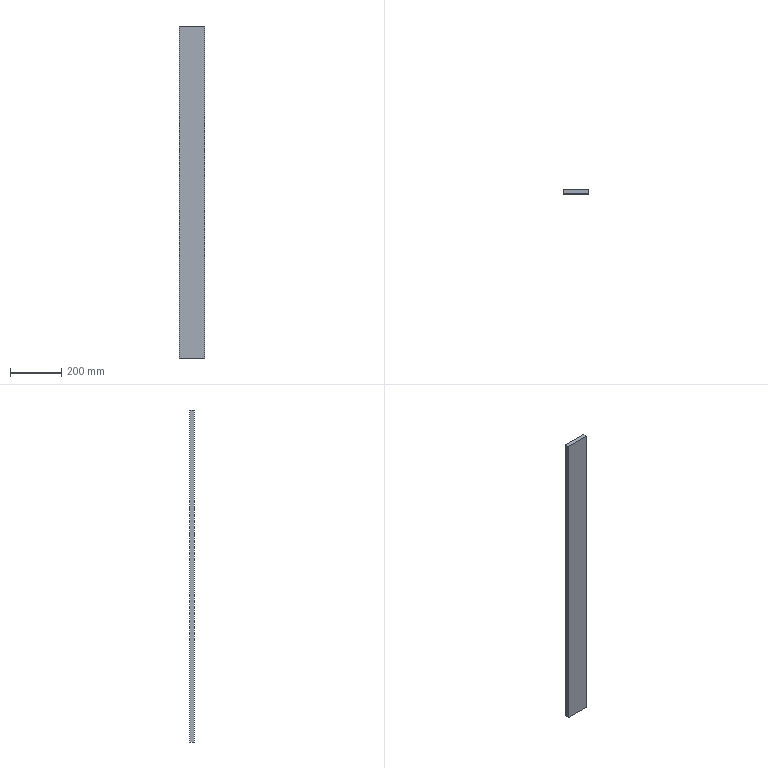Component | SolidWorks | GuideRailPad-1 | 1 solid | 6 faces | box 100 x 16 x 1300 mm | volume 2080000 mm3 | plane 6 | material Alloy Steel
build123d program:
from build123d import *

# Parameters (mm, degrees)
SKETCH1_W           = 100
SKETCH1_H           = 16
BOSS_EXTRUDE1_DEPTH = 650


with BuildPart() as part:
    # Sketch1 → Boss-Extrude1 (new, symmetric)
    with BuildSketch(Plane.XY):
        Rectangle(SKETCH1_W, SKETCH1_H)
    extrude(amount=BOSS_EXTRUDE1_DEPTH, both=True)


solid = part.part

# Placed as in the assembly
solid = solid.moved(Location((-7.456, -260.275, 1030), (0, 0, 0)))
STEP:
#1=COLOUR_RGB('',0.7922,0.8196,0.9333);
#2=FILL_AREA_STYLE_COLOUR('',#1);
#3=FILL_AREA_STYLE('',(#2));
#4=SURFACE_STYLE_FILL_AREA(#3);
#5=SURFACE_SIDE_STYLE('',(#4));
#6=SURFACE_STYLE_USAGE(.BOTH.,#5);
#7=PRESENTATION_STYLE_ASSIGNMENT((#6));
#8=CARTESIAN_POINT('',(-2.262,-9.932,14.961));
#9=VERTEX_POINT('',#8);
#10=CARTESIAN_POINT('',(-2.262,-10.562,14.961));
#11=VERTEX_POINT('',#10);
#12=CARTESIAN_POINT('',(-2.262,-10.562,14.961));
#13=DIRECTION('',(0.,-1.,0.));
#14=VECTOR('',#13,39.37);
#15=LINE('',#12,#14);
#16=EDGE_CURVE('',#9,#11,#15,.T.);
#17=ORIENTED_EDGE('',*,*,#16,.T.);
#18=CARTESIAN_POINT('',(-2.262,-10.562,66.142));
#19=VERTEX_POINT('',#18);
#20=CARTESIAN_POINT('',(-2.262,-10.562,66.142));
#21=DIRECTION('',(0.,0.,-1.));
#22=VECTOR('',#21,39.37);
#23=LINE('',#20,#22);
#24=EDGE_CURVE('',#19,#11,#23,.T.);
#25=ORIENTED_EDGE('',*,*,#24,.F.);
#26=CARTESIAN_POINT('',(-2.262,-9.932,66.142));
#27=VERTEX_POINT('',#26);
#28=CARTESIAN_POINT('',(-2.262,-10.562,66.142));
#29=DIRECTION('',(0.,-1.,0.));
#30=VECTOR('',#29,39.37);
#31=LINE('',#28,#30);
#32=EDGE_CURVE('',#27,#19,#31,.T.);
#33=ORIENTED_EDGE('',*,*,#32,.F.);
#34=CARTESIAN_POINT('',(-2.262,-9.932,66.142));
#35=DIRECTION('',(0.,0.,-1.));
#36=VECTOR('',#35,39.37);
#37=LINE('',#34,#36);
#38=EDGE_CURVE('',#27,#9,#37,.T.);
#39=ORIENTED_EDGE('',*,*,#38,.T.);
#40=EDGE_LOOP('',(#17,#25,#33,#39));
#41=FACE_OUTER_BOUND('',#40,.T.);
#42=CARTESIAN_POINT('',(-2.262,-10.562,66.142));
#43=DIRECTION('',(1.,0.,0.));
#44=DIRECTION('',(0.,0.,-1.));
#45=AXIS2_PLACEMENT_3D('',#42,#43,#44);
#46=PLANE('',#45);
#47=ADVANCED_FACE('',(#41),#46,.F.);
#48=CARTESIAN_POINT('',(1.675,-10.562,14.961));
#49=VERTEX_POINT('',#48);
#50=CARTESIAN_POINT('',(1.675,-10.562,14.961));
#51=DIRECTION('',(1.,0.,0.));
#52=VECTOR('',#51,39.37);
#53=LINE('',#50,#52);
#54=EDGE_CURVE('',#11,#49,#53,.T.);
#55=ORIENTED_EDGE('',*,*,#54,.T.);
#56=CARTESIAN_POINT('',(1.675,-10.562,66.142));
#57=VERTEX_POINT('',#56);
#58=CARTESIAN_POINT('',(1.675,-10.562,66.142));
#59=DIRECTION('',(0.,0.,-1.));
#60=VECTOR('',#59,39.37);
#61=LINE('',#58,#60);
#62=EDGE_CURVE('',#57,#49,#61,.T.);
#63=ORIENTED_EDGE('',*,*,#62,.F.);
#64=CARTESIAN_POINT('',(1.675,-10.562,66.142));
#65=DIRECTION('',(1.,0.,0.));
#66=VECTOR('',#65,39.37);
#67=LINE('',#64,#66);
#68=EDGE_CURVE('',#19,#57,#67,.T.);
#69=ORIENTED_EDGE('',*,*,#68,.F.);
#70=ORIENTED_EDGE('',*,*,#24,.T.);
#71=EDGE_LOOP('',(#55,#63,#69,#70));
#72=FACE_OUTER_BOUND('',#71,.T.);
#73=CARTESIAN_POINT('',(1.675,-10.562,66.142));
#74=DIRECTION('',(-0.,1.,0.));
#75=DIRECTION('',(-1.,-0.,0.));
#76=AXIS2_PLACEMENT_3D('',#73,#74,#75);
#77=PLANE('',#76);
#78=ADVANCED_FACE('',(#72),#77,.F.);
#79=CARTESIAN_POINT('',(1.675,-9.932,14.961));
#80=VERTEX_POINT('',#79);
#81=CARTESIAN_POINT('',(1.675,-10.562,14.961));
#82=DIRECTION('',(0.,1.,0.));
#83=VECTOR('',#82,39.37);
#84=LINE('',#81,#83);
#85=EDGE_CURVE('',#49,#80,#84,.T.);
#86=ORIENTED_EDGE('',*,*,#85,.T.);
#87=CARTESIAN_POINT('',(1.675,-9.932,66.142));
#88=VERTEX_POINT('',#87);
#89=CARTESIAN_POINT('',(1.675,-9.932,66.142));
#90=DIRECTION('',(0.,0.,-1.));
#91=VECTOR('',#90,39.37);
#92=LINE('',#89,#91);
#93=EDGE_CURVE('',#88,#80,#92,.T.);
#94=ORIENTED_EDGE('',*,*,#93,.F.);
#95=CARTESIAN_POINT('',(1.675,-10.562,66.142));
#96=DIRECTION('',(0.,1.,0.));
#97=VECTOR('',#96,39.37);
#98=LINE('',#95,#97);
#99=EDGE_CURVE('',#57,#88,#98,.T.);
#100=ORIENTED_EDGE('',*,*,#99,.F.);
#101=ORIENTED_EDGE('',*,*,#62,.T.);
#102=EDGE_LOOP('',(#86,#94,#100,#101));
#103=FACE_OUTER_BOUND('',#102,.T.);
#104=CARTESIAN_POINT('',(1.675,-10.562,66.142));
#105=DIRECTION('',(-1.,0.,0.));
#106=DIRECTION('',(0.,0.,1.));
#107=AXIS2_PLACEMENT_3D('',#104,#105,#106);
#108=PLANE('',#107);
#109=ADVANCED_FACE('',(#103),#108,.F.);
#110=CARTESIAN_POINT('',(1.675,-9.932,14.961));
#111=DIRECTION('',(-1.,-0.,0.));
#112=VECTOR('',#111,39.37);
#113=LINE('',#110,#112);
#114=EDGE_CURVE('',#80,#9,#113,.T.);
#115=ORIENTED_EDGE('',*,*,#114,.T.);
#116=ORIENTED_EDGE('',*,*,#38,.F.);
#117=CARTESIAN_POINT('',(1.675,-9.932,66.142));
#118=DIRECTION('',(-1.,-0.,0.));
#119=VECTOR('',#118,39.37);
#120=LINE('',#117,#119);
#121=EDGE_CURVE('',#88,#27,#120,.T.);
#122=ORIENTED_EDGE('',*,*,#121,.F.);
#123=ORIENTED_EDGE('',*,*,#93,.T.);
#124=EDGE_LOOP('',(#115,#116,#122,#123));
#125=FACE_OUTER_BOUND('',#124,.T.);
#126=CARTESIAN_POINT('',(1.675,-9.932,66.142));
#127=DIRECTION('',(0.,-1.,0.));
#128=DIRECTION('',(1.,0.,0.));
#129=AXIS2_PLACEMENT_3D('',#126,#127,#128);
#130=PLANE('',#129);
#131=ADVANCED_FACE('',(#125),#130,.F.);
#132=ORIENTED_EDGE('',*,*,#32,.T.);
#133=ORIENTED_EDGE('',*,*,#68,.T.);
#134=ORIENTED_EDGE('',*,*,#99,.T.);
#135=ORIENTED_EDGE('',*,*,#121,.T.);
#136=EDGE_LOOP('',(#132,#133,#134,#135));
#137=FACE_OUTER_BOUND('',#136,.T.);
#138=CARTESIAN_POINT('',(-2.262,-9.932,66.142));
#139=DIRECTION('',(0.,0.,1.));
#140=DIRECTION('',(1.,0.,0.));
#141=AXIS2_PLACEMENT_3D('',#138,#139,#140);
#142=PLANE('',#141);
#143=ADVANCED_FACE('',(#137),#142,.T.);
#144=ORIENTED_EDGE('',*,*,#16,.F.);
#145=ORIENTED_EDGE('',*,*,#114,.F.);
#146=ORIENTED_EDGE('',*,*,#85,.F.);
#147=ORIENTED_EDGE('',*,*,#54,.F.);
#148=EDGE_LOOP('',(#144,#145,#146,#147));
#149=FACE_OUTER_BOUND('',#148,.T.);
#150=CARTESIAN_POINT('',(-2.262,-9.932,14.961));
#151=DIRECTION('',(0.,0.,1.));
#152=DIRECTION('',(1.,0.,0.));
#153=AXIS2_PLACEMENT_3D('',#150,#151,#152);
#154=PLANE('',#153);
#155=ADVANCED_FACE('',(#149),#154,.F.);
#156=CLOSED_SHELL('',(#47,#78,#109,#131,#143,#155));
#157=MANIFOLD_SOLID_BREP('',#156);
#158=STYLED_ITEM('',(#7),#157);
#159=PRESENTATION_LAYER_ASSIGNMENT('','',(#158));
#160=(LENGTH_UNIT()NAMED_UNIT(*)SI_UNIT($,.METRE.));
#161=LENGTH_MEASURE_WITH_UNIT(LENGTH_MEASURE(0.0254),#160);
#162=DIMENSIONAL_EXPONENTS(1.,0.,0.,0.,0.,0.,0.);
#163=(CONVERSION_BASED_UNIT('',#161)LENGTH_UNIT()NAMED_UNIT(#162));
#164=UNCERTAINTY_MEASURE_WITH_UNIT(LENGTH_MEASURE(0.00001),#163,'','');
#165=(NAMED_UNIT(*)PLANE_ANGLE_UNIT()SI_UNIT($,.RADIAN.));
#166=(NAMED_UNIT(*)SI_UNIT($,.STERADIAN.)SOLID_ANGLE_UNIT());
#167=(GEOMETRIC_REPRESENTATION_CONTEXT(3)GLOBAL_UNCERTAINTY_ASSIGNED_CONTEXT((#164))GLOBAL_UNIT_ASSIGNED_CONTEXT((#163,#165,#166))REPRESENTATION_CONTEXT('',''));
#168=MECHANICAL_DESIGN_GEOMETRIC_PRESENTATION_REPRESENTATION('',(#158),#167);
#169=CARTESIAN_POINT('',(0.,0.,0.));
#170=DIRECTION('',(0.,0.,1.));
#171=DIRECTION('',(1.,0.,0.));
#172=AXIS2_PLACEMENT_3D('',#169,#170,#171);
#173=(LENGTH_UNIT()NAMED_UNIT(*)SI_UNIT($,.METRE.));
#174=LENGTH_MEASURE_WITH_UNIT(LENGTH_MEASURE(0.0254),#173);
#175=DIMENSIONAL_EXPONENTS(1.,0.,0.,0.,0.,0.,0.);
#176=(CONVERSION_BASED_UNIT('',#174)LENGTH_UNIT()NAMED_UNIT(#175));
#177=UNCERTAINTY_MEASURE_WITH_UNIT(LENGTH_MEASURE(0.00001),#176,'','');
#178=(NAMED_UNIT(*)PLANE_ANGLE_UNIT()SI_UNIT($,.RADIAN.));
#179=(NAMED_UNIT(*)SI_UNIT($,.STERADIAN.)SOLID_ANGLE_UNIT());
#180=(GEOMETRIC_REPRESENTATION_CONTEXT(3)GLOBAL_UNCERTAINTY_ASSIGNED_CONTEXT((#177))GLOBAL_UNIT_ASSIGNED_CONTEXT((#176,#178,#179))REPRESENTATION_CONTEXT('',''));
#181=ADVANCED_BREP_SHAPE_REPRESENTATION('',(#157,#172),#180);